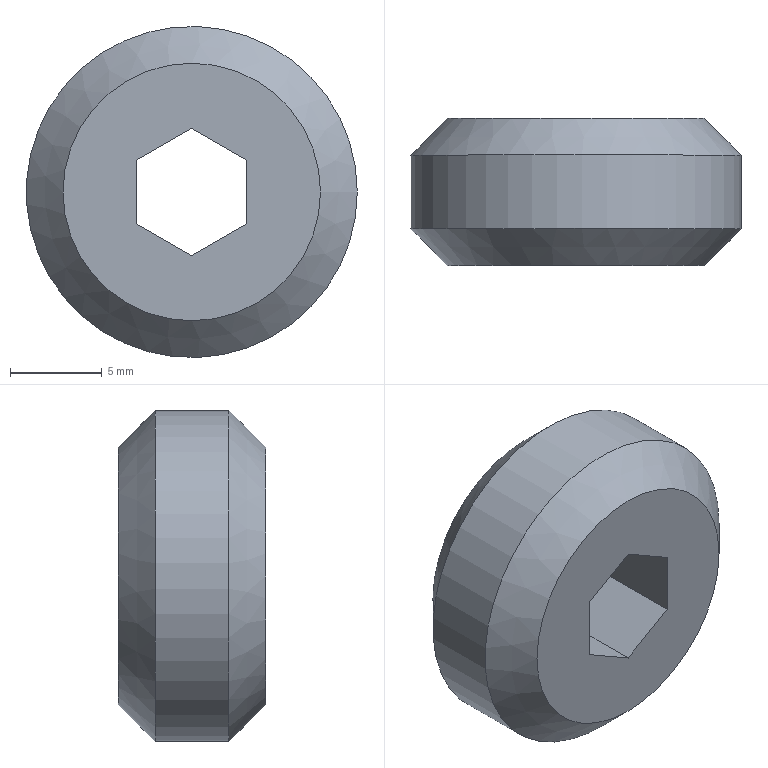Component | NX | ADJ_NUT | 1 solid | 11 faces | box 18 x 8 x 18 mm | volume 1577 mm3 | plane 8 | cone 2 | cylinder 1 | commonest cylinder face diameters 18 x1
STEP:
#1=CARTESIAN_POINT('',(0.,0.,0.));
#2=DIRECTION('',(0.,0.,1.));
#3=DIRECTION('',(1.,0.,0.));
#4=AXIS2_PLACEMENT_3D('',#1,#2,#3);
#5=CARTESIAN_POINT('',(40.195,115.209,-1.732));
#6=VERTEX_POINT('',#5);
#7=CARTESIAN_POINT('',(40.195,115.209,1.732));
#8=VERTEX_POINT('',#7);
#9=CARTESIAN_POINT('',(40.195,115.209,-1.732));
#10=DIRECTION('',(0.,0.,1.));
#11=VECTOR('',#10,1.);
#12=LINE('',#9,#11);
#13=CARTESIAN_POINT('',(40.195,107.209,-1.732));
#14=DIRECTION('',(-1.,0.,0.));
#15=DIRECTION('',(0.,-1.,0.));
#16=AXIS2_PLACEMENT_3D('',#13,#14,#15);
#17=PLANE('',#16);
#18=CARTESIAN_POINT('',(-8.,0.));
#19=DIRECTION('',(0.,1.));
#20=VECTOR('',#19,1.);
#21=LINE('',#18,#20);
#22=(GEOMETRIC_REPRESENTATION_CONTEXT(2)PARAMETRIC_REPRESENTATION_CONTEXT()REPRESENTATION_CONTEXT('',''));
#23=DEFINITIONAL_REPRESENTATION('',(#21),#22);
#24=PCURVE('',#17,#23);
#25=CARTESIAN_POINT('',(43.195,115.209,0.));
#26=DIRECTION('',(0.,-1.,0.));
#27=DIRECTION('',(1.,0.,0.));
#28=AXIS2_PLACEMENT_3D('',#25,#26,#27);
#29=PLANE('',#28);
#30=CARTESIAN_POINT('',(-3.,-1.732));
#31=DIRECTION('',(0.,1.));
#32=VECTOR('',#31,1.);
#33=LINE('',#30,#32);
#34=(GEOMETRIC_REPRESENTATION_CONTEXT(2)PARAMETRIC_REPRESENTATION_CONTEXT()REPRESENTATION_CONTEXT('',''));
#35=DEFINITIONAL_REPRESENTATION('',(#33),#34);
#36=PCURVE('',#29,#35);
#37=SURFACE_CURVE('',#12,(#24,#36),.PCURVE_S1.);
#38=EDGE_CURVE('',#6,#8,#37,.T.);
#39=ORIENTED_EDGE('',*,*,#38,.T.);
#40=CARTESIAN_POINT('',(40.195,107.209,1.732));
#41=VERTEX_POINT('',#40);
#42=CARTESIAN_POINT('',(40.195,107.209,1.732));
#43=DIRECTION('',(0.,1.,0.));
#44=VECTOR('',#43,1.);
#45=LINE('',#42,#44);
#46=CARTESIAN_POINT('',(0.,3.464));
#47=DIRECTION('',(-1.,0.));
#48=VECTOR('',#47,1.);
#49=LINE('',#46,#48);
#50=(GEOMETRIC_REPRESENTATION_CONTEXT(2)PARAMETRIC_REPRESENTATION_CONTEXT()REPRESENTATION_CONTEXT('',''));
#51=DEFINITIONAL_REPRESENTATION('',(#49),#50);
#52=PCURVE('',#17,#51);
#53=CARTESIAN_POINT('',(40.195,107.209,1.732));
#54=DIRECTION('',(-0.5,0.,0.866));
#55=DIRECTION('',(-0.866,0.,-0.5));
#56=AXIS2_PLACEMENT_3D('',#53,#54,#55);
#57=PLANE('',#56);
#58=CARTESIAN_POINT('',(0.,0.));
#59=DIRECTION('',(0.,-1.));
#60=VECTOR('',#59,1.);
#61=LINE('',#58,#60);
#62=(GEOMETRIC_REPRESENTATION_CONTEXT(2)PARAMETRIC_REPRESENTATION_CONTEXT()REPRESENTATION_CONTEXT('',''));
#63=DEFINITIONAL_REPRESENTATION('',(#61),#62);
#64=PCURVE('',#57,#63);
#65=SURFACE_CURVE('',#45,(#52,#64),.PCURVE_S1.);
#66=EDGE_CURVE('',#41,#8,#65,.T.);
#67=ORIENTED_EDGE('',*,*,#66,.F.);
#68=CARTESIAN_POINT('',(40.195,107.209,-1.732));
#69=VERTEX_POINT('',#68);
#70=CARTESIAN_POINT('',(40.195,107.209,-1.732));
#71=DIRECTION('',(0.,0.,1.));
#72=VECTOR('',#71,1.);
#73=LINE('',#70,#72);
#74=CARTESIAN_POINT('',(0.,0.));
#75=DIRECTION('',(0.,1.));
#76=VECTOR('',#75,1.);
#77=LINE('',#74,#76);
#78=(GEOMETRIC_REPRESENTATION_CONTEXT(2)PARAMETRIC_REPRESENTATION_CONTEXT()REPRESENTATION_CONTEXT('',''));
#79=DEFINITIONAL_REPRESENTATION('',(#77),#78);
#80=PCURVE('',#17,#79);
#81=CARTESIAN_POINT('',(43.195,107.209,0.));
#82=DIRECTION('',(0.,-1.,0.));
#83=DIRECTION('',(1.,0.,0.));
#84=AXIS2_PLACEMENT_3D('',#81,#82,#83);
#85=PLANE('',#84);
#86=CARTESIAN_POINT('',(-3.,-1.732));
#87=DIRECTION('',(0.,1.));
#88=VECTOR('',#87,1.);
#89=LINE('',#86,#88);
#90=(GEOMETRIC_REPRESENTATION_CONTEXT(2)PARAMETRIC_REPRESENTATION_CONTEXT()REPRESENTATION_CONTEXT('',''));
#91=DEFINITIONAL_REPRESENTATION('',(#89),#90);
#92=PCURVE('',#85,#91);
#93=SURFACE_CURVE('',#73,(#80,#92),.PCURVE_S1.);
#94=EDGE_CURVE('',#69,#41,#93,.T.);
#95=ORIENTED_EDGE('',*,*,#94,.F.);
#96=CARTESIAN_POINT('',(40.195,107.209,-1.732));
#97=DIRECTION('',(0.,1.,0.));
#98=VECTOR('',#97,1.);
#99=LINE('',#96,#98);
#100=CARTESIAN_POINT('',(0.,0.));
#101=DIRECTION('',(-1.,0.));
#102=VECTOR('',#101,1.);
#103=LINE('',#100,#102);
#104=(GEOMETRIC_REPRESENTATION_CONTEXT(2)PARAMETRIC_REPRESENTATION_CONTEXT()REPRESENTATION_CONTEXT('',''));
#105=DEFINITIONAL_REPRESENTATION('',(#103),#104);
#106=PCURVE('',#17,#105);
#107=CARTESIAN_POINT('',(43.195,107.209,-3.464));
#108=DIRECTION('',(-0.5,0.,-0.866));
#109=DIRECTION('',(0.866,0.,-0.5));
#110=AXIS2_PLACEMENT_3D('',#107,#108,#109);
#111=PLANE('',#110);
#112=CARTESIAN_POINT('',(-3.464,0.));
#113=DIRECTION('',(0.,-1.));
#114=VECTOR('',#113,1.);
#115=LINE('',#112,#114);
#116=(GEOMETRIC_REPRESENTATION_CONTEXT(2)PARAMETRIC_REPRESENTATION_CONTEXT()REPRESENTATION_CONTEXT('',''));
#117=DEFINITIONAL_REPRESENTATION('',(#115),#116);
#118=PCURVE('',#111,#117);
#119=SURFACE_CURVE('',#99,(#106,#118),.PCURVE_S1.);
#120=EDGE_CURVE('',#69,#6,#119,.T.);
#121=ORIENTED_EDGE('',*,*,#120,.T.);
#122=EDGE_LOOP('',(#39,#67,#95,#121));
#123=FACE_BOUND('',#122,.T.);
#124=ADVANCED_FACE('',(#123),#17,.F.);
#125=CARTESIAN_POINT('',(43.195,115.209,3.464));
#126=VERTEX_POINT('',#125);
#127=CARTESIAN_POINT('',(40.195,115.209,1.732));
#128=DIRECTION('',(0.866,0.,0.5));
#129=VECTOR('',#128,1.);
#130=LINE('',#127,#129);
#131=CARTESIAN_POINT('',(0.,-8.));
#132=DIRECTION('',(-1.,0.));
#133=VECTOR('',#132,1.);
#134=LINE('',#131,#133);
#135=(GEOMETRIC_REPRESENTATION_CONTEXT(2)PARAMETRIC_REPRESENTATION_CONTEXT()REPRESENTATION_CONTEXT('',''));
#136=DEFINITIONAL_REPRESENTATION('',(#134),#135);
#137=PCURVE('',#57,#136);
#138=CARTESIAN_POINT('',(-3.,1.732));
#139=DIRECTION('',(0.866,0.5));
#140=VECTOR('',#139,1.);
#141=LINE('',#138,#140);
#142=(GEOMETRIC_REPRESENTATION_CONTEXT(2)PARAMETRIC_REPRESENTATION_CONTEXT()REPRESENTATION_CONTEXT('',''));
#143=DEFINITIONAL_REPRESENTATION('',(#141),#142);
#144=PCURVE('',#29,#143);
#145=SURFACE_CURVE('',#130,(#137,#144),.PCURVE_S1.);
#146=EDGE_CURVE('',#8,#126,#145,.T.);
#147=ORIENTED_EDGE('',*,*,#146,.T.);
#148=CARTESIAN_POINT('',(43.195,107.209,3.464));
#149=VERTEX_POINT('',#148);
#150=CARTESIAN_POINT('',(43.195,107.209,3.464));
#151=DIRECTION('',(0.,1.,0.));
#152=VECTOR('',#151,1.);
#153=LINE('',#150,#152);
#154=CARTESIAN_POINT('',(-3.464,0.));
#155=DIRECTION('',(0.,-1.));
#156=VECTOR('',#155,1.);
#157=LINE('',#154,#156);
#158=(GEOMETRIC_REPRESENTATION_CONTEXT(2)PARAMETRIC_REPRESENTATION_CONTEXT()REPRESENTATION_CONTEXT('',''));
#159=DEFINITIONAL_REPRESENTATION('',(#157),#158);
#160=PCURVE('',#57,#159);
#161=CARTESIAN_POINT('',(43.195,107.209,3.464));
#162=DIRECTION('',(0.5,0.,0.866));
#163=DIRECTION('',(-0.866,0.,0.5));
#164=AXIS2_PLACEMENT_3D('',#161,#162,#163);
#165=PLANE('',#164);
#166=CARTESIAN_POINT('',(0.,0.));
#167=DIRECTION('',(0.,-1.));
#168=VECTOR('',#167,1.);
#169=LINE('',#166,#168);
#170=(GEOMETRIC_REPRESENTATION_CONTEXT(2)PARAMETRIC_REPRESENTATION_CONTEXT()REPRESENTATION_CONTEXT('',''));
#171=DEFINITIONAL_REPRESENTATION('',(#169),#170);
#172=PCURVE('',#165,#171);
#173=SURFACE_CURVE('',#153,(#160,#172),.PCURVE_S1.);
#174=EDGE_CURVE('',#149,#126,#173,.T.);
#175=ORIENTED_EDGE('',*,*,#174,.F.);
#176=CARTESIAN_POINT('',(40.195,107.209,1.732));
#177=DIRECTION('',(0.866,0.,0.5));
#178=VECTOR('',#177,1.);
#179=LINE('',#176,#178);
#180=CARTESIAN_POINT('',(0.,0.));
#181=DIRECTION('',(-1.,0.));
#182=VECTOR('',#181,1.);
#183=LINE('',#180,#182);
#184=(GEOMETRIC_REPRESENTATION_CONTEXT(2)PARAMETRIC_REPRESENTATION_CONTEXT()REPRESENTATION_CONTEXT('',''));
#185=DEFINITIONAL_REPRESENTATION('',(#183),#184);
#186=PCURVE('',#57,#185);
#187=CARTESIAN_POINT('',(-3.,1.732));
#188=DIRECTION('',(0.866,0.5));
#189=VECTOR('',#188,1.);
#190=LINE('',#187,#189);
#191=(GEOMETRIC_REPRESENTATION_CONTEXT(2)PARAMETRIC_REPRESENTATION_CONTEXT()REPRESENTATION_CONTEXT('',''));
#192=DEFINITIONAL_REPRESENTATION('',(#190),#191);
#193=PCURVE('',#85,#192);
#194=SURFACE_CURVE('',#179,(#186,#193),.PCURVE_S1.);
#195=EDGE_CURVE('',#41,#149,#194,.T.);
#196=ORIENTED_EDGE('',*,*,#195,.F.);
#197=ORIENTED_EDGE('',*,*,#66,.T.);
#198=EDGE_LOOP('',(#147,#175,#196,#197));
#199=FACE_BOUND('',#198,.T.);
#200=ADVANCED_FACE('',(#199),#57,.F.);
#201=CARTESIAN_POINT('',(46.195,115.209,1.732));
#202=VERTEX_POINT('',#201);
#203=CARTESIAN_POINT('',(43.195,115.209,3.464));
#204=DIRECTION('',(0.866,0.,-0.5));
#205=VECTOR('',#204,1.);
#206=LINE('',#203,#205);
#207=CARTESIAN_POINT('',(0.,-8.));
#208=DIRECTION('',(-1.,0.));
#209=VECTOR('',#208,1.);
#210=LINE('',#207,#209);
#211=(GEOMETRIC_REPRESENTATION_CONTEXT(2)PARAMETRIC_REPRESENTATION_CONTEXT()REPRESENTATION_CONTEXT('',''));
#212=DEFINITIONAL_REPRESENTATION('',(#210),#211);
#213=PCURVE('',#165,#212);
#214=CARTESIAN_POINT('',(0.,3.464));
#215=DIRECTION('',(0.866,-0.5));
#216=VECTOR('',#215,1.);
#217=LINE('',#214,#216);
#218=(GEOMETRIC_REPRESENTATION_CONTEXT(2)PARAMETRIC_REPRESENTATION_CONTEXT()REPRESENTATION_CONTEXT('',''));
#219=DEFINITIONAL_REPRESENTATION('',(#217),#218);
#220=PCURVE('',#29,#219);
#221=SURFACE_CURVE('',#206,(#213,#220),.PCURVE_S1.);
#222=EDGE_CURVE('',#126,#202,#221,.T.);
#223=ORIENTED_EDGE('',*,*,#222,.T.);
#224=CARTESIAN_POINT('',(46.195,107.209,1.732));
#225=VERTEX_POINT('',#224);
#226=CARTESIAN_POINT('',(46.195,107.209,1.732));
#227=DIRECTION('',(0.,1.,0.));
#228=VECTOR('',#227,1.);
#229=LINE('',#226,#228);
#230=CARTESIAN_POINT('',(-3.464,0.));
#231=DIRECTION('',(0.,-1.));
#232=VECTOR('',#231,1.);
#233=LINE('',#230,#232);
#234=(GEOMETRIC_REPRESENTATION_CONTEXT(2)PARAMETRIC_REPRESENTATION_CONTEXT()REPRESENTATION_CONTEXT('',''));
#235=DEFINITIONAL_REPRESENTATION('',(#233),#234);
#236=PCURVE('',#165,#235);
#237=CARTESIAN_POINT('',(46.195,107.209,1.732));
#238=DIRECTION('',(1.,0.,0.));
#239=DIRECTION('',(0.,1.,0.));
#240=AXIS2_PLACEMENT_3D('',#237,#238,#239);
#241=PLANE('',#240);
#242=CARTESIAN_POINT('',(0.,-0.));
#243=DIRECTION('',(1.,0.));
#244=VECTOR('',#243,1.);
#245=LINE('',#242,#244);
#246=(GEOMETRIC_REPRESENTATION_CONTEXT(2)PARAMETRIC_REPRESENTATION_CONTEXT()REPRESENTATION_CONTEXT('',''));
#247=DEFINITIONAL_REPRESENTATION('',(#245),#246);
#248=PCURVE('',#241,#247);
#249=SURFACE_CURVE('',#229,(#236,#248),.PCURVE_S1.);
#250=EDGE_CURVE('',#225,#202,#249,.T.);
#251=ORIENTED_EDGE('',*,*,#250,.F.);
#252=CARTESIAN_POINT('',(43.195,107.209,3.464));
#253=DIRECTION('',(0.866,0.,-0.5));
#254=VECTOR('',#253,1.);
#255=LINE('',#252,#254);
#256=CARTESIAN_POINT('',(0.,0.));
#257=DIRECTION('',(-1.,0.));
#258=VECTOR('',#257,1.);
#259=LINE('',#256,#258);
#260=(GEOMETRIC_REPRESENTATION_CONTEXT(2)PARAMETRIC_REPRESENTATION_CONTEXT()REPRESENTATION_CONTEXT('',''));
#261=DEFINITIONAL_REPRESENTATION('',(#259),#260);
#262=PCURVE('',#165,#261);
#263=CARTESIAN_POINT('',(0.,3.464));
#264=DIRECTION('',(0.866,-0.5));
#265=VECTOR('',#264,1.);
#266=LINE('',#263,#265);
#267=(GEOMETRIC_REPRESENTATION_CONTEXT(2)PARAMETRIC_REPRESENTATION_CONTEXT()REPRESENTATION_CONTEXT('',''));
#268=DEFINITIONAL_REPRESENTATION('',(#266),#267);
#269=PCURVE('',#85,#268);
#270=SURFACE_CURVE('',#255,(#262,#269),.PCURVE_S1.);
#271=EDGE_CURVE('',#149,#225,#270,.T.);
#272=ORIENTED_EDGE('',*,*,#271,.F.);
#273=ORIENTED_EDGE('',*,*,#174,.T.);
#274=EDGE_LOOP('',(#223,#251,#272,#273));
#275=FACE_BOUND('',#274,.T.);
#276=ADVANCED_FACE('',(#275),#165,.F.);
#277=CARTESIAN_POINT('',(46.195,115.209,-1.732));
#278=VERTEX_POINT('',#277);
#279=CARTESIAN_POINT('',(46.195,115.209,1.732));
#280=DIRECTION('',(0.,0.,-1.));
#281=VECTOR('',#280,1.);
#282=LINE('',#279,#281);
#283=CARTESIAN_POINT('',(8.,0.));
#284=DIRECTION('',(0.,-1.));
#285=VECTOR('',#284,1.);
#286=LINE('',#283,#285);
#287=(GEOMETRIC_REPRESENTATION_CONTEXT(2)PARAMETRIC_REPRESENTATION_CONTEXT()REPRESENTATION_CONTEXT('',''));
#288=DEFINITIONAL_REPRESENTATION('',(#286),#287);
#289=PCURVE('',#241,#288);
#290=CARTESIAN_POINT('',(3.,1.732));
#291=DIRECTION('',(0.,-1.));
#292=VECTOR('',#291,1.);
#293=LINE('',#290,#292);
#294=(GEOMETRIC_REPRESENTATION_CONTEXT(2)PARAMETRIC_REPRESENTATION_CONTEXT()REPRESENTATION_CONTEXT('',''));
#295=DEFINITIONAL_REPRESENTATION('',(#293),#294);
#296=PCURVE('',#29,#295);
#297=SURFACE_CURVE('',#282,(#289,#296),.PCURVE_S1.);
#298=EDGE_CURVE('',#202,#278,#297,.T.);
#299=ORIENTED_EDGE('',*,*,#298,.T.);
#300=CARTESIAN_POINT('',(46.195,107.209,-1.732));
#301=VERTEX_POINT('',#300);
#302=CARTESIAN_POINT('',(46.195,107.209,-1.732));
#303=DIRECTION('',(0.,1.,0.));
#304=VECTOR('',#303,1.);
#305=LINE('',#302,#304);
#306=CARTESIAN_POINT('',(0.,-3.464));
#307=DIRECTION('',(1.,0.));
#308=VECTOR('',#307,1.);
#309=LINE('',#306,#308);
#310=(GEOMETRIC_REPRESENTATION_CONTEXT(2)PARAMETRIC_REPRESENTATION_CONTEXT()REPRESENTATION_CONTEXT('',''));
#311=DEFINITIONAL_REPRESENTATION('',(#309),#310);
#312=PCURVE('',#241,#311);
#313=CARTESIAN_POINT('',(46.195,107.209,-1.732));
#314=DIRECTION('',(0.5,0.,-0.866));
#315=DIRECTION('',(0.866,0.,0.5));
#316=AXIS2_PLACEMENT_3D('',#313,#314,#315);
#317=PLANE('',#316);
#318=CARTESIAN_POINT('',(0.,0.));
#319=DIRECTION('',(0.,-1.));
#320=VECTOR('',#319,1.);
#321=LINE('',#318,#320);
#322=(GEOMETRIC_REPRESENTATION_CONTEXT(2)PARAMETRIC_REPRESENTATION_CONTEXT()REPRESENTATION_CONTEXT('',''));
#323=DEFINITIONAL_REPRESENTATION('',(#321),#322);
#324=PCURVE('',#317,#323);
#325=SURFACE_CURVE('',#305,(#312,#324),.PCURVE_S1.);
#326=EDGE_CURVE('',#301,#278,#325,.T.);
#327=ORIENTED_EDGE('',*,*,#326,.F.);
#328=CARTESIAN_POINT('',(46.195,107.209,1.732));
#329=DIRECTION('',(0.,0.,-1.));
#330=VECTOR('',#329,1.);
#331=LINE('',#328,#330);
#332=CARTESIAN_POINT('',(0.,0.));
#333=DIRECTION('',(0.,-1.));
#334=VECTOR('',#333,1.);
#335=LINE('',#332,#334);
#336=(GEOMETRIC_REPRESENTATION_CONTEXT(2)PARAMETRIC_REPRESENTATION_CONTEXT()REPRESENTATION_CONTEXT('',''));
#337=DEFINITIONAL_REPRESENTATION('',(#335),#336);
#338=PCURVE('',#241,#337);
#339=CARTESIAN_POINT('',(3.,1.732));
#340=DIRECTION('',(0.,-1.));
#341=VECTOR('',#340,1.);
#342=LINE('',#339,#341);
#343=(GEOMETRIC_REPRESENTATION_CONTEXT(2)PARAMETRIC_REPRESENTATION_CONTEXT()REPRESENTATION_CONTEXT('',''));
#344=DEFINITIONAL_REPRESENTATION('',(#342),#343);
#345=PCURVE('',#85,#344);
#346=SURFACE_CURVE('',#331,(#338,#345),.PCURVE_S1.);
#347=EDGE_CURVE('',#225,#301,#346,.T.);
#348=ORIENTED_EDGE('',*,*,#347,.F.);
#349=ORIENTED_EDGE('',*,*,#250,.T.);
#350=EDGE_LOOP('',(#299,#327,#348,#349));
#351=FACE_BOUND('',#350,.T.);
#352=ADVANCED_FACE('',(#351),#241,.F.);
#353=CARTESIAN_POINT('',(43.195,115.209,-3.464));
#354=VERTEX_POINT('',#353);
#355=CARTESIAN_POINT('',(46.195,115.209,-1.732));
#356=DIRECTION('',(-0.866,0.,-0.5));
#357=VECTOR('',#356,1.);
#358=LINE('',#355,#357);
#359=CARTESIAN_POINT('',(0.,-8.));
#360=DIRECTION('',(-1.,0.));
#361=VECTOR('',#360,1.);
#362=LINE('',#359,#361);
#363=(GEOMETRIC_REPRESENTATION_CONTEXT(2)PARAMETRIC_REPRESENTATION_CONTEXT()REPRESENTATION_CONTEXT('',''));
#364=DEFINITIONAL_REPRESENTATION('',(#362),#363);
#365=PCURVE('',#317,#364);
#366=CARTESIAN_POINT('',(3.,-1.732));
#367=DIRECTION('',(-0.866,-0.5));
#368=VECTOR('',#367,1.);
#369=LINE('',#366,#368);
#370=(GEOMETRIC_REPRESENTATION_CONTEXT(2)PARAMETRIC_REPRESENTATION_CONTEXT()REPRESENTATION_CONTEXT('',''));
#371=DEFINITIONAL_REPRESENTATION('',(#369),#370);
#372=PCURVE('',#29,#371);
#373=SURFACE_CURVE('',#358,(#365,#372),.PCURVE_S1.);
#374=EDGE_CURVE('',#278,#354,#373,.T.);
#375=ORIENTED_EDGE('',*,*,#374,.T.);
#376=CARTESIAN_POINT('',(43.195,107.209,-3.464));
#377=VERTEX_POINT('',#376);
#378=CARTESIAN_POINT('',(43.195,107.209,-3.464));
#379=DIRECTION('',(0.,1.,0.));
#380=VECTOR('',#379,1.);
#381=LINE('',#378,#380);
#382=CARTESIAN_POINT('',(-3.464,0.));
#383=DIRECTION('',(0.,-1.));
#384=VECTOR('',#383,1.);
#385=LINE('',#382,#384);
#386=(GEOMETRIC_REPRESENTATION_CONTEXT(2)PARAMETRIC_REPRESENTATION_CONTEXT()REPRESENTATION_CONTEXT('',''));
#387=DEFINITIONAL_REPRESENTATION('',(#385),#386);
#388=PCURVE('',#317,#387);
#389=CARTESIAN_POINT('',(0.,0.));
#390=DIRECTION('',(0.,-1.));
#391=VECTOR('',#390,1.);
#392=LINE('',#389,#391);
#393=(GEOMETRIC_REPRESENTATION_CONTEXT(2)PARAMETRIC_REPRESENTATION_CONTEXT()REPRESENTATION_CONTEXT('',''));
#394=DEFINITIONAL_REPRESENTATION('',(#392),#393);
#395=PCURVE('',#111,#394);
#396=SURFACE_CURVE('',#381,(#388,#395),.PCURVE_S1.);
#397=EDGE_CURVE('',#377,#354,#396,.T.);
#398=ORIENTED_EDGE('',*,*,#397,.F.);
#399=CARTESIAN_POINT('',(46.195,107.209,-1.732));
#400=DIRECTION('',(-0.866,0.,-0.5));
#401=VECTOR('',#400,1.);
#402=LINE('',#399,#401);
#403=CARTESIAN_POINT('',(0.,0.));
#404=DIRECTION('',(-1.,0.));
#405=VECTOR('',#404,1.);
#406=LINE('',#403,#405);
#407=(GEOMETRIC_REPRESENTATION_CONTEXT(2)PARAMETRIC_REPRESENTATION_CONTEXT()REPRESENTATION_CONTEXT('',''));
#408=DEFINITIONAL_REPRESENTATION('',(#406),#407);
#409=PCURVE('',#317,#408);
#410=CARTESIAN_POINT('',(3.,-1.732));
#411=DIRECTION('',(-0.866,-0.5));
#412=VECTOR('',#411,1.);
#413=LINE('',#410,#412);
#414=(GEOMETRIC_REPRESENTATION_CONTEXT(2)PARAMETRIC_REPRESENTATION_CONTEXT()REPRESENTATION_CONTEXT('',''));
#415=DEFINITIONAL_REPRESENTATION('',(#413),#414);
#416=PCURVE('',#85,#415);
#417=SURFACE_CURVE('',#402,(#409,#416),.PCURVE_S1.);
#418=EDGE_CURVE('',#301,#377,#417,.T.);
#419=ORIENTED_EDGE('',*,*,#418,.F.);
#420=ORIENTED_EDGE('',*,*,#326,.T.);
#421=EDGE_LOOP('',(#375,#398,#419,#420));
#422=FACE_BOUND('',#421,.T.);
#423=ADVANCED_FACE('',(#422),#317,.F.);
#424=CARTESIAN_POINT('',(52.195,113.209,0.));
#425=VERTEX_POINT('',#424);
#426=CARTESIAN_POINT('',(43.195,113.209,0.));
#427=DIRECTION('',(0.,-1.,0.));
#428=DIRECTION('',(1.,0.,0.));
#429=AXIS2_PLACEMENT_3D('',#426,#427,#428);
#430=CIRCLE('',#429,9.);
#431=CARTESIAN_POINT('',(43.195,107.209,0.));
#432=DIRECTION('',(0.,1.,0.));
#433=DIRECTION('',(-1.,0.,0.));
#434=AXIS2_PLACEMENT_3D('',#431,#432,#433);
#435=CYLINDRICAL_SURFACE('',#434,9.);
#436=CARTESIAN_POINT('',(9.425,6.));
#437=DIRECTION('',(-1.,0.));
#438=VECTOR('',#437,1.);
#439=LINE('',#436,#438);
#440=(GEOMETRIC_REPRESENTATION_CONTEXT(2)PARAMETRIC_REPRESENTATION_CONTEXT()REPRESENTATION_CONTEXT('',''));
#441=DEFINITIONAL_REPRESENTATION('',(#439),#440);
#442=PCURVE('',#435,#441);
#443=CARTESIAN_POINT('',(43.195,113.209,0.));
#444=DIRECTION('',(0.,-1.,0.));
#445=DIRECTION('',(1.,0.,0.));
#446=AXIS2_PLACEMENT_3D('',#443,#444,#445);
#447=CONICAL_SURFACE('',#446,9.,0.7854);
#448=CARTESIAN_POINT('',(0.,0.));
#449=DIRECTION('',(1.,0.));
#450=VECTOR('',#449,1.);
#451=LINE('',#448,#450);
#452=(GEOMETRIC_REPRESENTATION_CONTEXT(2)PARAMETRIC_REPRESENTATION_CONTEXT()REPRESENTATION_CONTEXT('',''));
#453=DEFINITIONAL_REPRESENTATION('',(#451),#452);
#454=PCURVE('',#447,#453);
#455=SURFACE_CURVE('',#430,(#442,#454),.PCURVE_S1.);
#456=EDGE_CURVE('',#425,#425,#455,.T.);
#457=ORIENTED_EDGE('',*,*,#456,.T.);
#458=CARTESIAN_POINT('',(52.195,109.209,0.));
#459=VERTEX_POINT('',#458);
#460=CARTESIAN_POINT('',(52.195,109.209,0.));
#461=CARTESIAN_POINT('',(52.195,113.209,0.));
#462=B_SPLINE_CURVE_WITH_KNOTS('',1,(#460,#461),.UNSPECIFIED.,.F.,.F.,(2,2),(2.,6.),.PIECEWISE_BEZIER_KNOTS.);
#463=CARTESIAN_POINT('',(3.142,0.));
#464=DIRECTION('',(0.,1.));
#465=VECTOR('',#464,1.);
#466=LINE('',#463,#465);
#467=(GEOMETRIC_REPRESENTATION_CONTEXT(2)PARAMETRIC_REPRESENTATION_CONTEXT()REPRESENTATION_CONTEXT('',''));
#468=DEFINITIONAL_REPRESENTATION('',(#466),#467);
#469=PCURVE('',#435,#468);
#470=CARTESIAN_POINT('',(9.425,0.));
#471=DIRECTION('',(0.,1.));
#472=VECTOR('',#471,1.);
#473=LINE('',#470,#472);
#474=(GEOMETRIC_REPRESENTATION_CONTEXT(2)PARAMETRIC_REPRESENTATION_CONTEXT()REPRESENTATION_CONTEXT('',''));
#475=DEFINITIONAL_REPRESENTATION('',(#473),#474);
#476=PCURVE('',#435,#475);
#477=SEAM_CURVE('',#462,(#469,#476),.PCURVE_S1.);
#478=EDGE_CURVE('',#459,#425,#477,.T.);
#479=ORIENTED_EDGE('',*,*,#478,.F.);
#480=CARTESIAN_POINT('',(43.195,109.209,0.));
#481=DIRECTION('',(0.,1.,0.));
#482=DIRECTION('',(1.,0.,0.));
#483=AXIS2_PLACEMENT_3D('',#480,#481,#482);
#484=CIRCLE('',#483,9.);
#485=CARTESIAN_POINT('',(3.142,2.));
#486=DIRECTION('',(1.,0.));
#487=VECTOR('',#486,1.);
#488=LINE('',#485,#487);
#489=(GEOMETRIC_REPRESENTATION_CONTEXT(2)PARAMETRIC_REPRESENTATION_CONTEXT()REPRESENTATION_CONTEXT('',''));
#490=DEFINITIONAL_REPRESENTATION('',(#488),#489);
#491=PCURVE('',#435,#490);
#492=CARTESIAN_POINT('',(43.195,107.209,0.));
#493=DIRECTION('',(0.,1.,0.));
#494=DIRECTION('',(-1.,0.,0.));
#495=AXIS2_PLACEMENT_3D('',#492,#493,#494);
#496=CONICAL_SURFACE('',#495,7.,0.7854);
#497=CARTESIAN_POINT('',(3.142,2.));
#498=DIRECTION('',(1.,0.));
#499=VECTOR('',#498,1.);
#500=LINE('',#497,#499);
#501=(GEOMETRIC_REPRESENTATION_CONTEXT(2)PARAMETRIC_REPRESENTATION_CONTEXT()REPRESENTATION_CONTEXT('',''));
#502=DEFINITIONAL_REPRESENTATION('',(#500),#501);
#503=PCURVE('',#496,#502);
#504=SURFACE_CURVE('',#484,(#491,#503),.PCURVE_S1.);
#505=EDGE_CURVE('',#459,#459,#504,.T.);
#506=ORIENTED_EDGE('',*,*,#505,.T.);
#507=ORIENTED_EDGE('',*,*,#478,.T.);
#508=EDGE_LOOP('',(#457,#479,#506,#507));
#509=FACE_BOUND('',#508,.T.);
#510=ADVANCED_FACE('',(#509),#435,.T.);
#511=CARTESIAN_POINT('',(43.195,115.209,-3.464));
#512=DIRECTION('',(-0.866,0.,0.5));
#513=VECTOR('',#512,1.);
#514=LINE('',#511,#513);
#515=CARTESIAN_POINT('',(0.,-8.));
#516=DIRECTION('',(-1.,0.));
#517=VECTOR('',#516,1.);
#518=LINE('',#515,#517);
#519=(GEOMETRIC_REPRESENTATION_CONTEXT(2)PARAMETRIC_REPRESENTATION_CONTEXT()REPRESENTATION_CONTEXT('',''));
#520=DEFINITIONAL_REPRESENTATION('',(#518),#519);
#521=PCURVE('',#111,#520);
#522=CARTESIAN_POINT('',(0.,-3.464));
#523=DIRECTION('',(-0.866,0.5));
#524=VECTOR('',#523,1.);
#525=LINE('',#522,#524);
#526=(GEOMETRIC_REPRESENTATION_CONTEXT(2)PARAMETRIC_REPRESENTATION_CONTEXT()REPRESENTATION_CONTEXT('',''));
#527=DEFINITIONAL_REPRESENTATION('',(#525),#526);
#528=PCURVE('',#29,#527);
#529=SURFACE_CURVE('',#514,(#521,#528),.PCURVE_S1.);
#530=EDGE_CURVE('',#354,#6,#529,.T.);
#531=ORIENTED_EDGE('',*,*,#530,.T.);
#532=ORIENTED_EDGE('',*,*,#120,.F.);
#533=CARTESIAN_POINT('',(43.195,107.209,-3.464));
#534=DIRECTION('',(-0.866,0.,0.5));
#535=VECTOR('',#534,1.);
#536=LINE('',#533,#535);
#537=CARTESIAN_POINT('',(0.,0.));
#538=DIRECTION('',(-1.,0.));
#539=VECTOR('',#538,1.);
#540=LINE('',#537,#539);
#541=(GEOMETRIC_REPRESENTATION_CONTEXT(2)PARAMETRIC_REPRESENTATION_CONTEXT()REPRESENTATION_CONTEXT('',''));
#542=DEFINITIONAL_REPRESENTATION('',(#540),#541);
#543=PCURVE('',#111,#542);
#544=CARTESIAN_POINT('',(0.,-3.464));
#545=DIRECTION('',(-0.866,0.5));
#546=VECTOR('',#545,1.);
#547=LINE('',#544,#546);
#548=(GEOMETRIC_REPRESENTATION_CONTEXT(2)PARAMETRIC_REPRESENTATION_CONTEXT()REPRESENTATION_CONTEXT('',''));
#549=DEFINITIONAL_REPRESENTATION('',(#547),#548);
#550=PCURVE('',#85,#549);
#551=SURFACE_CURVE('',#536,(#543,#550),.PCURVE_S1.);
#552=EDGE_CURVE('',#377,#69,#551,.T.);
#553=ORIENTED_EDGE('',*,*,#552,.F.);
#554=ORIENTED_EDGE('',*,*,#397,.T.);
#555=EDGE_LOOP('',(#531,#532,#553,#554));
#556=FACE_BOUND('',#555,.T.);
#557=ADVANCED_FACE('',(#556),#111,.F.);
#558=CARTESIAN_POINT('',(50.195,107.209,0.));
#559=VERTEX_POINT('',#558);
#560=CARTESIAN_POINT('',(43.195,107.209,0.));
#561=DIRECTION('',(0.,-1.,0.));
#562=DIRECTION('',(1.,0.,0.));
#563=AXIS2_PLACEMENT_3D('',#560,#561,#562);
#564=CIRCLE('',#563,7.);
#565=CARTESIAN_POINT('',(0.,0.));
#566=DIRECTION('',(1.,0.));
#567=AXIS2_PLACEMENT_2D('',#565,#566);
#568=CIRCLE('',#567,7.);
#569=(GEOMETRIC_REPRESENTATION_CONTEXT(2)PARAMETRIC_REPRESENTATION_CONTEXT()REPRESENTATION_CONTEXT('',''));
#570=DEFINITIONAL_REPRESENTATION('',(#568),#569);
#571=PCURVE('',#85,#570);
#572=CARTESIAN_POINT('',(9.425,0.));
#573=DIRECTION('',(-1.,0.));
#574=VECTOR('',#573,1.);
#575=LINE('',#572,#574);
#576=(GEOMETRIC_REPRESENTATION_CONTEXT(2)PARAMETRIC_REPRESENTATION_CONTEXT()REPRESENTATION_CONTEXT('',''));
#577=DEFINITIONAL_REPRESENTATION('',(#575),#576);
#578=PCURVE('',#496,#577);
#579=SURFACE_CURVE('',#564,(#571,#578),.PCURVE_S1.);
#580=EDGE_CURVE('',#559,#559,#579,.T.);
#581=ORIENTED_EDGE('',*,*,#580,.T.);
#582=EDGE_LOOP('',(#581));
#583=FACE_BOUND('',#582,.T.);
#584=ORIENTED_EDGE('',*,*,#94,.T.);
#585=ORIENTED_EDGE('',*,*,#195,.T.);
#586=ORIENTED_EDGE('',*,*,#271,.T.);
#587=ORIENTED_EDGE('',*,*,#347,.T.);
#588=ORIENTED_EDGE('',*,*,#418,.T.);
#589=ORIENTED_EDGE('',*,*,#552,.T.);
#590=EDGE_LOOP('',(#584,#585,#586,#587,#588,#589));
#591=FACE_BOUND('',#590,.T.);
#592=ADVANCED_FACE('',(#583,#591),#85,.T.);
#593=CARTESIAN_POINT('',(50.195,115.209,0.));
#594=VERTEX_POINT('',#593);
#595=CARTESIAN_POINT('',(43.195,115.209,0.));
#596=DIRECTION('',(0.,1.,0.));
#597=DIRECTION('',(1.,0.,0.));
#598=AXIS2_PLACEMENT_3D('',#595,#596,#597);
#599=CIRCLE('',#598,7.);
#600=CARTESIAN_POINT('',(7.,0.));
#601=CARTESIAN_POINT('',(7.,-12.124));
#602=CARTESIAN_POINT('',(-3.5,-6.062));
#603=CARTESIAN_POINT('',(-14.,-0.));
#604=CARTESIAN_POINT('',(-3.5,6.062));
#605=CARTESIAN_POINT('',(7.,12.124));
#606=CARTESIAN_POINT('',(7.,0.));
#607=(BOUNDED_CURVE()B_SPLINE_CURVE(2,(#600,#601,#602,#603,#604,#605,#606),.UNSPECIFIED.,.T.,.F.)B_SPLINE_CURVE_WITH_KNOTS((1,2,2,2,2,1),(-2.094,0.,2.094,4.189,6.283,8.378),.UNSPECIFIED.)CURVE()GEOMETRIC_REPRESENTATION_ITEM()RATIONAL_B_SPLINE_CURVE((1.,0.5,1.,0.5,1.,0.5,1.))REPRESENTATION_ITEM(''));
#608=(GEOMETRIC_REPRESENTATION_CONTEXT(2)PARAMETRIC_REPRESENTATION_CONTEXT()REPRESENTATION_CONTEXT('',''));
#609=DEFINITIONAL_REPRESENTATION('',(#607),#608);
#610=PCURVE('',#29,#609);
#611=CARTESIAN_POINT('',(6.283,-2.));
#612=DIRECTION('',(-1.,0.));
#613=VECTOR('',#612,1.);
#614=LINE('',#611,#613);
#615=(GEOMETRIC_REPRESENTATION_CONTEXT(2)PARAMETRIC_REPRESENTATION_CONTEXT()REPRESENTATION_CONTEXT('',''));
#616=DEFINITIONAL_REPRESENTATION('',(#614),#615);
#617=PCURVE('',#447,#616);
#618=SURFACE_CURVE('',#599,(#610,#617),.PCURVE_S1.);
#619=EDGE_CURVE('',#594,#594,#618,.T.);
#620=ORIENTED_EDGE('',*,*,#619,.T.);
#621=EDGE_LOOP('',(#620));
#622=FACE_BOUND('',#621,.T.);
#623=ORIENTED_EDGE('',*,*,#38,.F.);
#624=ORIENTED_EDGE('',*,*,#530,.F.);
#625=ORIENTED_EDGE('',*,*,#374,.F.);
#626=ORIENTED_EDGE('',*,*,#298,.F.);
#627=ORIENTED_EDGE('',*,*,#222,.F.);
#628=ORIENTED_EDGE('',*,*,#146,.F.);
#629=EDGE_LOOP('',(#623,#624,#625,#626,#627,#628));
#630=FACE_BOUND('',#629,.T.);
#631=ADVANCED_FACE('',(#622,#630),#29,.F.);
#632=ORIENTED_EDGE('',*,*,#619,.F.);
#633=CARTESIAN_POINT('',(50.195,115.209,0.));
#634=CARTESIAN_POINT('',(52.195,113.209,0.));
#635=B_SPLINE_CURVE_WITH_KNOTS('',1,(#633,#634),.UNSPECIFIED.,.F.,.F.,(2,2),(-2.828,0.),.PIECEWISE_BEZIER_KNOTS.);
#636=CARTESIAN_POINT('',(6.283,0.));
#637=DIRECTION('',(0.,1.));
#638=VECTOR('',#637,1.);
#639=LINE('',#636,#638);
#640=(GEOMETRIC_REPRESENTATION_CONTEXT(2)PARAMETRIC_REPRESENTATION_CONTEXT()REPRESENTATION_CONTEXT('',''));
#641=DEFINITIONAL_REPRESENTATION('',(#639),#640);
#642=PCURVE('',#447,#641);
#643=CARTESIAN_POINT('',(0.,0.));
#644=DIRECTION('',(0.,1.));
#645=VECTOR('',#644,1.);
#646=LINE('',#643,#645);
#647=(GEOMETRIC_REPRESENTATION_CONTEXT(2)PARAMETRIC_REPRESENTATION_CONTEXT()REPRESENTATION_CONTEXT('',''));
#648=DEFINITIONAL_REPRESENTATION('',(#646),#647);
#649=PCURVE('',#447,#648);
#650=SEAM_CURVE('',#635,(#642,#649),.PCURVE_S1.);
#651=EDGE_CURVE('',#594,#425,#650,.T.);
#652=ORIENTED_EDGE('',*,*,#651,.T.);
#653=ORIENTED_EDGE('',*,*,#456,.F.);
#654=ORIENTED_EDGE('',*,*,#651,.F.);
#655=EDGE_LOOP('',(#632,#652,#653,#654));
#656=FACE_BOUND('',#655,.T.);
#657=ADVANCED_FACE('',(#656),#447,.T.);
#658=ORIENTED_EDGE('',*,*,#505,.F.);
#659=CARTESIAN_POINT('',(50.195,107.209,0.));
#660=CARTESIAN_POINT('',(52.195,109.209,0.));
#661=B_SPLINE_CURVE_WITH_KNOTS('',1,(#659,#660),.UNSPECIFIED.,.F.,.F.,(2,2),(0.,2.828),.PIECEWISE_BEZIER_KNOTS.);
#662=CARTESIAN_POINT('',(3.142,0.));
#663=DIRECTION('',(0.,1.));
#664=VECTOR('',#663,1.);
#665=LINE('',#662,#664);
#666=(GEOMETRIC_REPRESENTATION_CONTEXT(2)PARAMETRIC_REPRESENTATION_CONTEXT()REPRESENTATION_CONTEXT('',''));
#667=DEFINITIONAL_REPRESENTATION('',(#665),#666);
#668=PCURVE('',#496,#667);
#669=CARTESIAN_POINT('',(9.425,0.));
#670=DIRECTION('',(0.,1.));
#671=VECTOR('',#670,1.);
#672=LINE('',#669,#671);
#673=(GEOMETRIC_REPRESENTATION_CONTEXT(2)PARAMETRIC_REPRESENTATION_CONTEXT()REPRESENTATION_CONTEXT('',''));
#674=DEFINITIONAL_REPRESENTATION('',(#672),#673);
#675=PCURVE('',#496,#674);
#676=SEAM_CURVE('',#661,(#668,#675),.PCURVE_S1.);
#677=EDGE_CURVE('',#559,#459,#676,.T.);
#678=ORIENTED_EDGE('',*,*,#677,.F.);
#679=ORIENTED_EDGE('',*,*,#580,.F.);
#680=ORIENTED_EDGE('',*,*,#677,.T.);
#681=EDGE_LOOP('',(#658,#678,#679,#680));
#682=FACE_BOUND('',#681,.T.);
#683=ADVANCED_FACE('',(#682),#496,.T.);
#684=CLOSED_SHELL('',(#124,#200,#276,#352,#423,#510,#557,#592,#631,#657,#683));
#685=MANIFOLD_SOLID_BREP('',#684);
#686=(LENGTH_UNIT()NAMED_UNIT(*)SI_UNIT(.MILLI.,.METRE.));
#687=UNCERTAINTY_MEASURE_WITH_UNIT(LENGTH_MEASURE(0.000002),#686,'','');
#688=(NAMED_UNIT(*)PLANE_ANGLE_UNIT()SI_UNIT($,.RADIAN.));
#689=(NAMED_UNIT(*)SI_UNIT($,.STERADIAN.)SOLID_ANGLE_UNIT());
#690=(GEOMETRIC_REPRESENTATION_CONTEXT(3)GLOBAL_UNCERTAINTY_ASSIGNED_CONTEXT((#687))GLOBAL_UNIT_ASSIGNED_CONTEXT((#686,#688,#689))REPRESENTATION_CONTEXT('',''));
#691=ADVANCED_BREP_SHAPE_REPRESENTATION('',(#4,#685),#690);